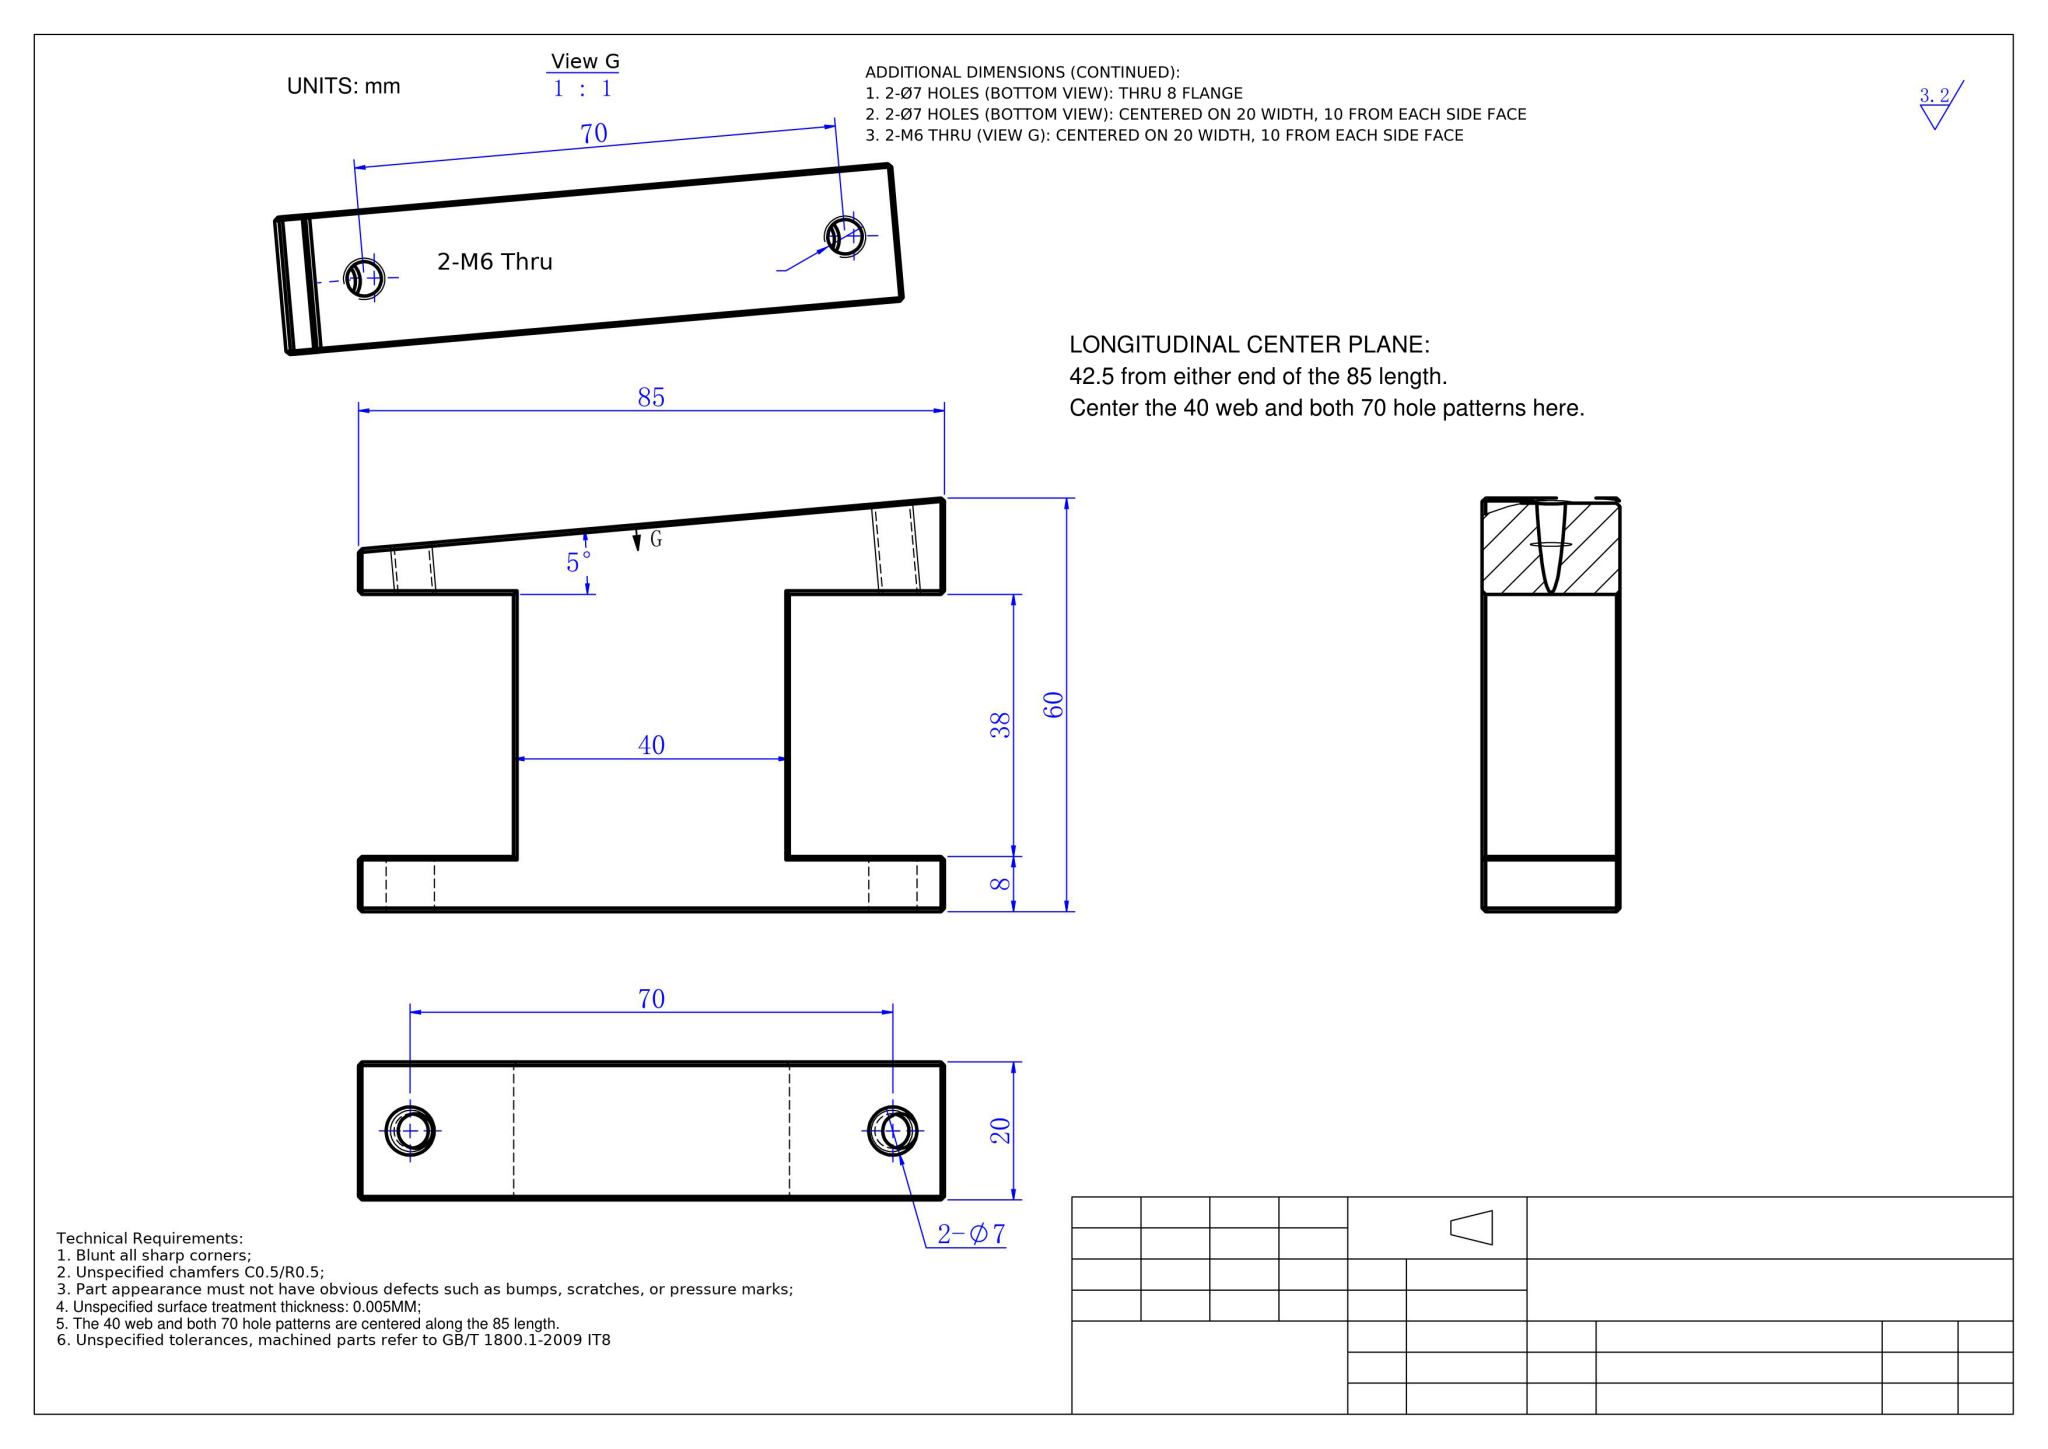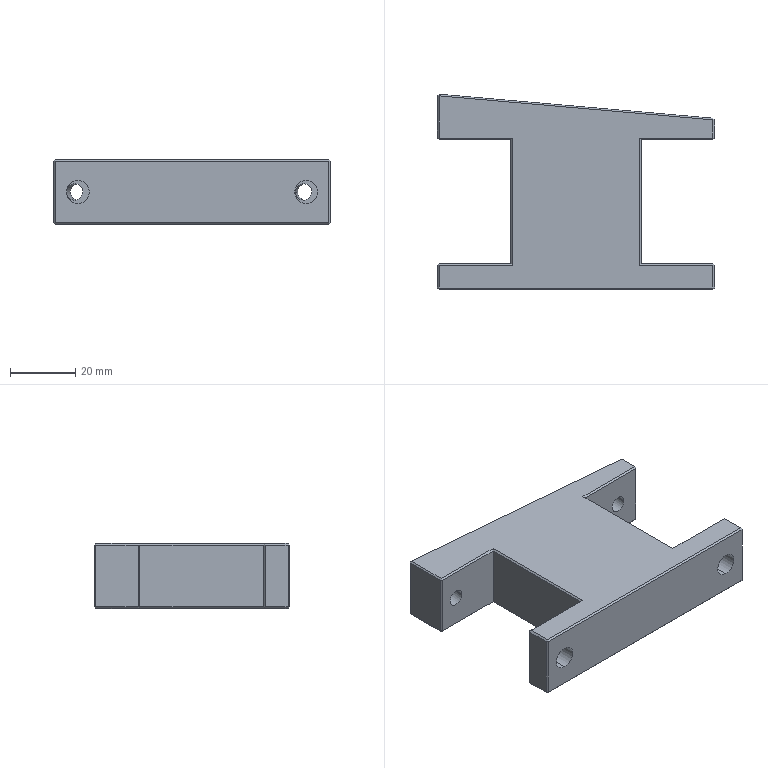Part | NX | mm | 1 solid | 70 faces | box 85 x 59.96 x 20 mm | volume 60346 mm3 | plane 62 | cylinder 8 | commonest cylinder face diameters 7 x4 5 x4